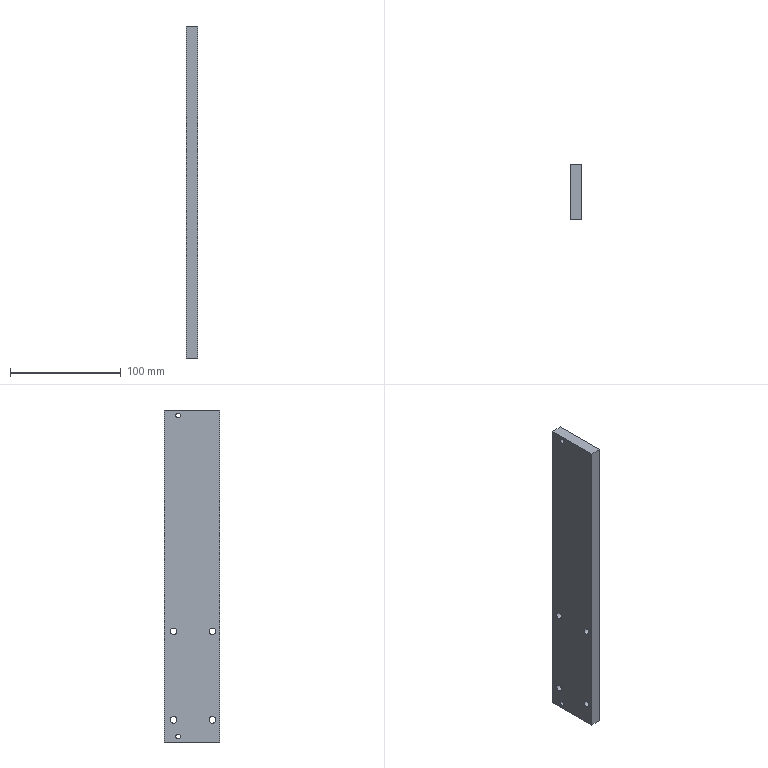Component | SolidWorks | ElectricalBoxAssembly2-1_GuidePlate-1 | 1 solid | 18 faces | box 10 x 50 x 300 mm | volume 148592 mm3 | cylinder 12 | plane 6 | commonest cylinder face diameters 6 x8 4.2 x4
build123d program:
from build123d import *

# Parameters (mm, degrees)
SKETCH1_W           = 300
SKETCH1_H           = 50
SKETCH1_R           = 3
BOSS_EXTRUDE1_DEPTH = 10
M5_TAPPED_HOLE1_D   = 4.2


with BuildPart() as part:
    # Sketch1 → Boss-Extrude1 (new body)
    with BuildSketch(Plane.XY):
        Rectangle(SKETCH1_W, SKETCH1_H)
        with Locations((130, 16.612)):
            Circle(SKETCH1_R, mode=Mode.SUBTRACT)
        with Locations((130, -18.388)):
            Circle(SKETCH1_R, mode=Mode.SUBTRACT)
        with Locations((50, 16.612)):
            Circle(SKETCH1_R, mode=Mode.SUBTRACT)
        with Locations((50, -18.388)):
            Circle(SKETCH1_R, mode=Mode.SUBTRACT)
    extrude(amount=BOSS_EXTRUDE1_DEPTH)

    # M5 Tapped Hole1 (through all)
    with Locations(Plane.XY.offset(10)):
        with Locations((-145, 12.5), (145, 12.5)):
            Hole(M5_TAPPED_HOLE1_D / 2)


solid = part.part

# Placed as in the assembly
solid = solid.moved(Location((745.468, 149.666, 1906.399), (0, 90, 0)))
STEP:
#1=COLOUR_RGB('',0.7922,0.8196,0.9333);
#2=FILL_AREA_STYLE_COLOUR('',#1);
#3=FILL_AREA_STYLE('',(#2));
#4=SURFACE_STYLE_FILL_AREA(#3);
#5=SURFACE_SIDE_STYLE('',(#4));
#6=SURFACE_STYLE_USAGE(.BOTH.,#5);
#7=PRESENTATION_STYLE_ASSIGNMENT((#6));
#8=CARTESIAN_POINT('',(29.349,6.384,80.846));
#9=VERTEX_POINT('',#8);
#10=CARTESIAN_POINT('',(29.349,6.384,80.681));
#11=VERTEX_POINT('',#10);
#12=CARTESIAN_POINT('',(29.349,6.384,80.764));
#13=DIRECTION('',(1.,-0.,0.));
#14=DIRECTION('',(0.,0.,-1.));
#15=AXIS2_PLACEMENT_3D('',#12,#13,#14);
#16=CIRCLE('',#15,0.08268);
#17=EDGE_CURVE('',#9,#11,#16,.T.);
#18=ORIENTED_EDGE('',*,*,#17,.F.);
#19=CARTESIAN_POINT('',(29.743,6.384,80.846));
#20=VERTEX_POINT('',#19);
#21=CARTESIAN_POINT('',(29.743,6.384,80.846));
#22=DIRECTION('',(1.,-0.,0.));
#23=VECTOR('',#22,39.37);
#24=LINE('',#21,#23);
#25=EDGE_CURVE('',#9,#20,#24,.T.);
#26=ORIENTED_EDGE('',*,*,#25,.T.);
#27=CARTESIAN_POINT('',(29.743,6.384,80.681));
#28=VERTEX_POINT('',#27);
#29=CARTESIAN_POINT('',(29.743,6.384,80.764));
#30=DIRECTION('',(1.,-0.,0.));
#31=DIRECTION('',(0.,0.,-1.));
#32=AXIS2_PLACEMENT_3D('',#29,#30,#31);
#33=CIRCLE('',#32,0.08268);
#34=EDGE_CURVE('',#20,#28,#33,.T.);
#35=ORIENTED_EDGE('',*,*,#34,.T.);
#36=CARTESIAN_POINT('',(29.743,6.384,80.681));
#37=DIRECTION('',(1.,-0.,0.));
#38=VECTOR('',#37,39.37);
#39=LINE('',#36,#38);
#40=EDGE_CURVE('',#11,#28,#39,.T.);
#41=ORIENTED_EDGE('',*,*,#40,.F.);
#42=EDGE_LOOP('',(#18,#26,#35,#41));
#43=FACE_OUTER_BOUND('',#42,.T.);
#44=CARTESIAN_POINT('',(29.743,6.384,80.764));
#45=DIRECTION('',(1.,-0.,0.));
#46=DIRECTION('',(0.,0.,-1.));
#47=AXIS2_PLACEMENT_3D('',#44,#45,#46);
#48=CYLINDRICAL_SURFACE('',#47,0.08268);
#49=ADVANCED_FACE('',(#43),#48,.F.);
#50=CARTESIAN_POINT('',(29.349,6.384,69.429));
#51=VERTEX_POINT('',#50);
#52=CARTESIAN_POINT('',(29.349,6.384,69.264));
#53=VERTEX_POINT('',#52);
#54=CARTESIAN_POINT('',(29.349,6.384,69.346));
#55=DIRECTION('',(1.,-0.,0.));
#56=DIRECTION('',(0.,0.,-1.));
#57=AXIS2_PLACEMENT_3D('',#54,#55,#56);
#58=CIRCLE('',#57,0.08268);
#59=EDGE_CURVE('',#51,#53,#58,.T.);
#60=ORIENTED_EDGE('',*,*,#59,.F.);
#61=CARTESIAN_POINT('',(29.743,6.384,69.429));
#62=VERTEX_POINT('',#61);
#63=CARTESIAN_POINT('',(29.743,6.384,69.429));
#64=DIRECTION('',(1.,-0.,0.));
#65=VECTOR('',#64,39.37);
#66=LINE('',#63,#65);
#67=EDGE_CURVE('',#51,#62,#66,.T.);
#68=ORIENTED_EDGE('',*,*,#67,.T.);
#69=CARTESIAN_POINT('',(29.743,6.384,69.264));
#70=VERTEX_POINT('',#69);
#71=CARTESIAN_POINT('',(29.743,6.384,69.346));
#72=DIRECTION('',(1.,-0.,0.));
#73=DIRECTION('',(0.,0.,-1.));
#74=AXIS2_PLACEMENT_3D('',#71,#72,#73);
#75=CIRCLE('',#74,0.08268);
#76=EDGE_CURVE('',#62,#70,#75,.T.);
#77=ORIENTED_EDGE('',*,*,#76,.T.);
#78=CARTESIAN_POINT('',(29.743,6.384,69.264));
#79=DIRECTION('',(1.,-0.,0.));
#80=VECTOR('',#79,39.37);
#81=LINE('',#78,#80);
#82=EDGE_CURVE('',#53,#70,#81,.T.);
#83=ORIENTED_EDGE('',*,*,#82,.F.);
#84=EDGE_LOOP('',(#60,#68,#77,#83));
#85=FACE_OUTER_BOUND('',#84,.T.);
#86=CARTESIAN_POINT('',(29.743,6.384,69.346));
#87=DIRECTION('',(1.,-0.,0.));
#88=DIRECTION('',(0.,0.,-1.));
#89=AXIS2_PLACEMENT_3D('',#86,#87,#88);
#90=CYLINDRICAL_SURFACE('',#89,0.08268);
#91=ADVANCED_FACE('',(#85),#90,.F.);
#92=CARTESIAN_POINT('',(29.743,5.168,73.205));
#93=VERTEX_POINT('',#92);
#94=CARTESIAN_POINT('',(29.743,5.168,72.968));
#95=VERTEX_POINT('',#94);
#96=CARTESIAN_POINT('',(29.743,5.168,73.087));
#97=DIRECTION('',(1.,-0.,0.));
#98=DIRECTION('',(0.,0.,-1.));
#99=AXIS2_PLACEMENT_3D('',#96,#97,#98);
#100=CIRCLE('',#99,0.1181);
#101=EDGE_CURVE('',#93,#95,#100,.T.);
#102=ORIENTED_EDGE('',*,*,#101,.T.);
#103=CARTESIAN_POINT('',(29.349,5.168,72.968));
#104=VERTEX_POINT('',#103);
#105=CARTESIAN_POINT('',(29.743,5.168,72.968));
#106=DIRECTION('',(-1.,0.,-0.));
#107=VECTOR('',#106,39.37);
#108=LINE('',#105,#107);
#109=EDGE_CURVE('',#95,#104,#108,.T.);
#110=ORIENTED_EDGE('',*,*,#109,.T.);
#111=CARTESIAN_POINT('',(29.349,5.168,73.205));
#112=VERTEX_POINT('',#111);
#113=CARTESIAN_POINT('',(29.349,5.168,73.087));
#114=DIRECTION('',(1.,-0.,0.));
#115=DIRECTION('',(0.,0.,-1.));
#116=AXIS2_PLACEMENT_3D('',#113,#114,#115);
#117=CIRCLE('',#116,0.1181);
#118=EDGE_CURVE('',#112,#104,#117,.T.);
#119=ORIENTED_EDGE('',*,*,#118,.F.);
#120=CARTESIAN_POINT('',(29.743,5.168,73.205));
#121=DIRECTION('',(-1.,0.,-0.));
#122=VECTOR('',#121,39.37);
#123=LINE('',#120,#122);
#124=EDGE_CURVE('',#93,#112,#123,.T.);
#125=ORIENTED_EDGE('',*,*,#124,.F.);
#126=EDGE_LOOP('',(#102,#110,#119,#125));
#127=FACE_OUTER_BOUND('',#126,.T.);
#128=CARTESIAN_POINT('',(29.743,5.168,73.087));
#129=DIRECTION('',(-1.,0.,-0.));
#130=DIRECTION('',(0.,0.,1.));
#131=AXIS2_PLACEMENT_3D('',#128,#129,#130);
#132=CYLINDRICAL_SURFACE('',#131,0.1181);
#133=ADVANCED_FACE('',(#127),#132,.F.);
#134=CARTESIAN_POINT('',(29.743,6.546,73.205));
#135=VERTEX_POINT('',#134);
#136=CARTESIAN_POINT('',(29.743,6.546,72.968));
#137=VERTEX_POINT('',#136);
#138=CARTESIAN_POINT('',(29.743,6.546,73.087));
#139=DIRECTION('',(1.,-0.,0.));
#140=DIRECTION('',(0.,0.,-1.));
#141=AXIS2_PLACEMENT_3D('',#138,#139,#140);
#142=CIRCLE('',#141,0.1181);
#143=EDGE_CURVE('',#135,#137,#142,.T.);
#144=ORIENTED_EDGE('',*,*,#143,.T.);
#145=CARTESIAN_POINT('',(29.349,6.546,72.968));
#146=VERTEX_POINT('',#145);
#147=CARTESIAN_POINT('',(29.743,6.546,72.968));
#148=DIRECTION('',(-1.,0.,-0.));
#149=VECTOR('',#148,39.37);
#150=LINE('',#147,#149);
#151=EDGE_CURVE('',#137,#146,#150,.T.);
#152=ORIENTED_EDGE('',*,*,#151,.T.);
#153=CARTESIAN_POINT('',(29.349,6.546,73.205));
#154=VERTEX_POINT('',#153);
#155=CARTESIAN_POINT('',(29.349,6.546,73.087));
#156=DIRECTION('',(1.,-0.,0.));
#157=DIRECTION('',(0.,0.,-1.));
#158=AXIS2_PLACEMENT_3D('',#155,#156,#157);
#159=CIRCLE('',#158,0.1181);
#160=EDGE_CURVE('',#154,#146,#159,.T.);
#161=ORIENTED_EDGE('',*,*,#160,.F.);
#162=CARTESIAN_POINT('',(29.743,6.546,73.205));
#163=DIRECTION('',(-1.,0.,-0.));
#164=VECTOR('',#163,39.37);
#165=LINE('',#162,#164);
#166=EDGE_CURVE('',#135,#154,#165,.T.);
#167=ORIENTED_EDGE('',*,*,#166,.F.);
#168=EDGE_LOOP('',(#144,#152,#161,#167));
#169=FACE_OUTER_BOUND('',#168,.T.);
#170=CARTESIAN_POINT('',(29.743,6.546,73.087));
#171=DIRECTION('',(-1.,0.,-0.));
#172=DIRECTION('',(0.,0.,1.));
#173=AXIS2_PLACEMENT_3D('',#170,#171,#172);
#174=CYLINDRICAL_SURFACE('',#173,0.1181);
#175=ADVANCED_FACE('',(#169),#174,.F.);
#176=CARTESIAN_POINT('',(29.743,5.168,70.055));
#177=VERTEX_POINT('',#176);
#178=CARTESIAN_POINT('',(29.743,5.168,69.819));
#179=VERTEX_POINT('',#178);
#180=CARTESIAN_POINT('',(29.743,5.168,69.937));
#181=DIRECTION('',(1.,-0.,0.));
#182=DIRECTION('',(0.,0.,-1.));
#183=AXIS2_PLACEMENT_3D('',#180,#181,#182);
#184=CIRCLE('',#183,0.1181);
#185=EDGE_CURVE('',#177,#179,#184,.T.);
#186=ORIENTED_EDGE('',*,*,#185,.T.);
#187=CARTESIAN_POINT('',(29.349,5.168,69.819));
#188=VERTEX_POINT('',#187);
#189=CARTESIAN_POINT('',(29.743,5.168,69.819));
#190=DIRECTION('',(-1.,0.,-0.));
#191=VECTOR('',#190,39.37);
#192=LINE('',#189,#191);
#193=EDGE_CURVE('',#179,#188,#192,.T.);
#194=ORIENTED_EDGE('',*,*,#193,.T.);
#195=CARTESIAN_POINT('',(29.349,5.168,70.055));
#196=VERTEX_POINT('',#195);
#197=CARTESIAN_POINT('',(29.349,5.168,69.937));
#198=DIRECTION('',(1.,-0.,0.));
#199=DIRECTION('',(0.,0.,-1.));
#200=AXIS2_PLACEMENT_3D('',#197,#198,#199);
#201=CIRCLE('',#200,0.1181);
#202=EDGE_CURVE('',#196,#188,#201,.T.);
#203=ORIENTED_EDGE('',*,*,#202,.F.);
#204=CARTESIAN_POINT('',(29.743,5.168,70.055));
#205=DIRECTION('',(-1.,0.,-0.));
#206=VECTOR('',#205,39.37);
#207=LINE('',#204,#206);
#208=EDGE_CURVE('',#177,#196,#207,.T.);
#209=ORIENTED_EDGE('',*,*,#208,.F.);
#210=EDGE_LOOP('',(#186,#194,#203,#209));
#211=FACE_OUTER_BOUND('',#210,.T.);
#212=CARTESIAN_POINT('',(29.743,5.168,69.937));
#213=DIRECTION('',(-1.,0.,-0.));
#214=DIRECTION('',(0.,0.,1.));
#215=AXIS2_PLACEMENT_3D('',#212,#213,#214);
#216=CYLINDRICAL_SURFACE('',#215,0.1181);
#217=ADVANCED_FACE('',(#211),#216,.F.);
#218=CARTESIAN_POINT('',(29.743,6.546,70.055));
#219=VERTEX_POINT('',#218);
#220=CARTESIAN_POINT('',(29.743,6.546,69.819));
#221=VERTEX_POINT('',#220);
#222=CARTESIAN_POINT('',(29.743,6.546,69.937));
#223=DIRECTION('',(1.,-0.,0.));
#224=DIRECTION('',(0.,0.,-1.));
#225=AXIS2_PLACEMENT_3D('',#222,#223,#224);
#226=CIRCLE('',#225,0.1181);
#227=EDGE_CURVE('',#219,#221,#226,.T.);
#228=ORIENTED_EDGE('',*,*,#227,.T.);
#229=CARTESIAN_POINT('',(29.349,6.546,69.819));
#230=VERTEX_POINT('',#229);
#231=CARTESIAN_POINT('',(29.743,6.546,69.819));
#232=DIRECTION('',(-1.,0.,-0.));
#233=VECTOR('',#232,39.37);
#234=LINE('',#231,#233);
#235=EDGE_CURVE('',#221,#230,#234,.T.);
#236=ORIENTED_EDGE('',*,*,#235,.T.);
#237=CARTESIAN_POINT('',(29.349,6.546,70.055));
#238=VERTEX_POINT('',#237);
#239=CARTESIAN_POINT('',(29.349,6.546,69.937));
#240=DIRECTION('',(1.,-0.,0.));
#241=DIRECTION('',(0.,0.,-1.));
#242=AXIS2_PLACEMENT_3D('',#239,#240,#241);
#243=CIRCLE('',#242,0.1181);
#244=EDGE_CURVE('',#238,#230,#243,.T.);
#245=ORIENTED_EDGE('',*,*,#244,.F.);
#246=CARTESIAN_POINT('',(29.743,6.546,70.055));
#247=DIRECTION('',(-1.,0.,-0.));
#248=VECTOR('',#247,39.37);
#249=LINE('',#246,#248);
#250=EDGE_CURVE('',#219,#238,#249,.T.);
#251=ORIENTED_EDGE('',*,*,#250,.F.);
#252=EDGE_LOOP('',(#228,#236,#245,#251));
#253=FACE_OUTER_BOUND('',#252,.T.);
#254=CARTESIAN_POINT('',(29.743,6.546,69.937));
#255=DIRECTION('',(-1.,0.,-0.));
#256=DIRECTION('',(0.,0.,1.));
#257=AXIS2_PLACEMENT_3D('',#254,#255,#256);
#258=CYLINDRICAL_SURFACE('',#257,0.1181);
#259=ADVANCED_FACE('',(#253),#258,.F.);
#260=CARTESIAN_POINT('',(29.743,6.384,80.764));
#261=DIRECTION('',(1.,-0.,0.));
#262=DIRECTION('',(0.,0.,-1.));
#263=AXIS2_PLACEMENT_3D('',#260,#261,#262);
#264=CIRCLE('',#263,0.08268);
#265=EDGE_CURVE('',#28,#20,#264,.T.);
#266=ORIENTED_EDGE('',*,*,#265,.F.);
#267=ORIENTED_EDGE('',*,*,#34,.F.);
#268=EDGE_LOOP('',(#266,#267));
#269=FACE_BOUND('',#268,.T.);
#270=CARTESIAN_POINT('',(29.743,6.384,69.346));
#271=DIRECTION('',(1.,-0.,0.));
#272=DIRECTION('',(0.,0.,-1.));
#273=AXIS2_PLACEMENT_3D('',#270,#271,#272);
#274=CIRCLE('',#273,0.08268);
#275=EDGE_CURVE('',#70,#62,#274,.T.);
#276=ORIENTED_EDGE('',*,*,#275,.F.);
#277=ORIENTED_EDGE('',*,*,#76,.F.);
#278=EDGE_LOOP('',(#276,#277));
#279=FACE_BOUND('',#278,.T.);
#280=ORIENTED_EDGE('',*,*,#143,.F.);
#281=CARTESIAN_POINT('',(29.743,6.546,73.087));
#282=DIRECTION('',(1.,-0.,0.));
#283=DIRECTION('',(0.,0.,-1.));
#284=AXIS2_PLACEMENT_3D('',#281,#282,#283);
#285=CIRCLE('',#284,0.1181);
#286=EDGE_CURVE('',#137,#135,#285,.T.);
#287=ORIENTED_EDGE('',*,*,#286,.F.);
#288=EDGE_LOOP('',(#280,#287));
#289=FACE_BOUND('',#288,.T.);
#290=ORIENTED_EDGE('',*,*,#227,.F.);
#291=CARTESIAN_POINT('',(29.743,6.546,69.937));
#292=DIRECTION('',(1.,-0.,0.));
#293=DIRECTION('',(0.,0.,-1.));
#294=AXIS2_PLACEMENT_3D('',#291,#292,#293);
#295=CIRCLE('',#294,0.1181);
#296=EDGE_CURVE('',#221,#219,#295,.T.);
#297=ORIENTED_EDGE('',*,*,#296,.F.);
#298=EDGE_LOOP('',(#290,#297));
#299=FACE_BOUND('',#298,.T.);
#300=CARTESIAN_POINT('',(29.743,4.908,69.15));
#301=VERTEX_POINT('',#300);
#302=CARTESIAN_POINT('',(29.743,6.877,69.15));
#303=VERTEX_POINT('',#302);
#304=CARTESIAN_POINT('',(29.743,6.877,69.15));
#305=DIRECTION('',(0.,1.,-0.));
#306=VECTOR('',#305,39.37);
#307=LINE('',#304,#306);
#308=EDGE_CURVE('',#301,#303,#307,.T.);
#309=ORIENTED_EDGE('',*,*,#308,.T.);
#310=CARTESIAN_POINT('',(29.743,6.877,80.961));
#311=VERTEX_POINT('',#310);
#312=CARTESIAN_POINT('',(29.743,6.877,80.961));
#313=DIRECTION('',(-0.,0.,1.));
#314=VECTOR('',#313,39.37);
#315=LINE('',#312,#314);
#316=EDGE_CURVE('',#303,#311,#315,.T.);
#317=ORIENTED_EDGE('',*,*,#316,.T.);
#318=CARTESIAN_POINT('',(29.743,4.908,80.961));
#319=VERTEX_POINT('',#318);
#320=CARTESIAN_POINT('',(29.743,6.877,80.961));
#321=DIRECTION('',(-0.,-1.,0.));
#322=VECTOR('',#321,39.37);
#323=LINE('',#320,#322);
#324=EDGE_CURVE('',#311,#319,#323,.T.);
#325=ORIENTED_EDGE('',*,*,#324,.T.);
#326=CARTESIAN_POINT('',(29.743,4.908,80.961));
#327=DIRECTION('',(0.,-0.,-1.));
#328=VECTOR('',#327,39.37);
#329=LINE('',#326,#328);
#330=EDGE_CURVE('',#319,#301,#329,.T.);
#331=ORIENTED_EDGE('',*,*,#330,.T.);
#332=EDGE_LOOP('',(#309,#317,#325,#331));
#333=FACE_OUTER_BOUND('',#332,.T.);
#334=ORIENTED_EDGE('',*,*,#185,.F.);
#335=CARTESIAN_POINT('',(29.743,5.168,69.937));
#336=DIRECTION('',(1.,-0.,0.));
#337=DIRECTION('',(0.,0.,-1.));
#338=AXIS2_PLACEMENT_3D('',#335,#336,#337);
#339=CIRCLE('',#338,0.1181);
#340=EDGE_CURVE('',#179,#177,#339,.T.);
#341=ORIENTED_EDGE('',*,*,#340,.F.);
#342=EDGE_LOOP('',(#334,#341));
#343=FACE_BOUND('',#342,.T.);
#344=ORIENTED_EDGE('',*,*,#101,.F.);
#345=CARTESIAN_POINT('',(29.743,5.168,73.087));
#346=DIRECTION('',(1.,-0.,0.));
#347=DIRECTION('',(0.,0.,-1.));
#348=AXIS2_PLACEMENT_3D('',#345,#346,#347);
#349=CIRCLE('',#348,0.1181);
#350=EDGE_CURVE('',#95,#93,#349,.T.);
#351=ORIENTED_EDGE('',*,*,#350,.F.);
#352=EDGE_LOOP('',(#344,#351));
#353=FACE_BOUND('',#352,.T.);
#354=CARTESIAN_POINT('',(29.743,5.892,75.055));
#355=DIRECTION('',(1.,-0.,0.));
#356=DIRECTION('',(0.,-0.,-1.));
#357=AXIS2_PLACEMENT_3D('',#354,#355,#356);
#358=PLANE('',#357);
#359=ADVANCED_FACE('',(#269,#279,#289,#299,#333,#343,#353),#358,.T.);
#360=CARTESIAN_POINT('',(29.349,6.384,80.764));
#361=DIRECTION('',(1.,-0.,0.));
#362=DIRECTION('',(0.,0.,-1.));
#363=AXIS2_PLACEMENT_3D('',#360,#361,#362);
#364=CIRCLE('',#363,0.08268);
#365=EDGE_CURVE('',#11,#9,#364,.T.);
#366=ORIENTED_EDGE('',*,*,#365,.T.);
#367=ORIENTED_EDGE('',*,*,#17,.T.);
#368=EDGE_LOOP('',(#366,#367));
#369=FACE_BOUND('',#368,.T.);
#370=CARTESIAN_POINT('',(29.349,6.384,69.346));
#371=DIRECTION('',(1.,-0.,0.));
#372=DIRECTION('',(0.,0.,-1.));
#373=AXIS2_PLACEMENT_3D('',#370,#371,#372);
#374=CIRCLE('',#373,0.08268);
#375=EDGE_CURVE('',#53,#51,#374,.T.);
#376=ORIENTED_EDGE('',*,*,#375,.T.);
#377=ORIENTED_EDGE('',*,*,#59,.T.);
#378=EDGE_LOOP('',(#376,#377));
#379=FACE_BOUND('',#378,.T.);
#380=CARTESIAN_POINT('',(29.349,4.908,69.15));
#381=VERTEX_POINT('',#380);
#382=CARTESIAN_POINT('',(29.349,6.877,69.15));
#383=VERTEX_POINT('',#382);
#384=CARTESIAN_POINT('',(29.349,6.877,69.15));
#385=DIRECTION('',(0.,1.,-0.));
#386=VECTOR('',#385,39.37);
#387=LINE('',#384,#386);
#388=EDGE_CURVE('',#381,#383,#387,.T.);
#389=ORIENTED_EDGE('',*,*,#388,.F.);
#390=CARTESIAN_POINT('',(29.349,4.908,80.961));
#391=VERTEX_POINT('',#390);
#392=CARTESIAN_POINT('',(29.349,4.908,80.961));
#393=DIRECTION('',(0.,-0.,-1.));
#394=VECTOR('',#393,39.37);
#395=LINE('',#392,#394);
#396=EDGE_CURVE('',#391,#381,#395,.T.);
#397=ORIENTED_EDGE('',*,*,#396,.F.);
#398=CARTESIAN_POINT('',(29.349,6.877,80.961));
#399=VERTEX_POINT('',#398);
#400=CARTESIAN_POINT('',(29.349,6.877,80.961));
#401=DIRECTION('',(-0.,-1.,0.));
#402=VECTOR('',#401,39.37);
#403=LINE('',#400,#402);
#404=EDGE_CURVE('',#399,#391,#403,.T.);
#405=ORIENTED_EDGE('',*,*,#404,.F.);
#406=CARTESIAN_POINT('',(29.349,6.877,80.961));
#407=DIRECTION('',(-0.,0.,1.));
#408=VECTOR('',#407,39.37);
#409=LINE('',#406,#408);
#410=EDGE_CURVE('',#383,#399,#409,.T.);
#411=ORIENTED_EDGE('',*,*,#410,.F.);
#412=EDGE_LOOP('',(#389,#397,#405,#411));
#413=FACE_OUTER_BOUND('',#412,.T.);
#414=ORIENTED_EDGE('',*,*,#244,.T.);
#415=CARTESIAN_POINT('',(29.349,6.546,69.937));
#416=DIRECTION('',(1.,-0.,0.));
#417=DIRECTION('',(0.,0.,-1.));
#418=AXIS2_PLACEMENT_3D('',#415,#416,#417);
#419=CIRCLE('',#418,0.1181);
#420=EDGE_CURVE('',#230,#238,#419,.T.);
#421=ORIENTED_EDGE('',*,*,#420,.T.);
#422=EDGE_LOOP('',(#414,#421));
#423=FACE_BOUND('',#422,.T.);
#424=ORIENTED_EDGE('',*,*,#202,.T.);
#425=CARTESIAN_POINT('',(29.349,5.168,69.937));
#426=DIRECTION('',(1.,-0.,0.));
#427=DIRECTION('',(0.,0.,-1.));
#428=AXIS2_PLACEMENT_3D('',#425,#426,#427);
#429=CIRCLE('',#428,0.1181);
#430=EDGE_CURVE('',#188,#196,#429,.T.);
#431=ORIENTED_EDGE('',*,*,#430,.T.);
#432=EDGE_LOOP('',(#424,#431));
#433=FACE_BOUND('',#432,.T.);
#434=ORIENTED_EDGE('',*,*,#160,.T.);
#435=CARTESIAN_POINT('',(29.349,6.546,73.087));
#436=DIRECTION('',(1.,-0.,0.));
#437=DIRECTION('',(0.,0.,-1.));
#438=AXIS2_PLACEMENT_3D('',#435,#436,#437);
#439=CIRCLE('',#438,0.1181);
#440=EDGE_CURVE('',#146,#154,#439,.T.);
#441=ORIENTED_EDGE('',*,*,#440,.T.);
#442=EDGE_LOOP('',(#434,#441));
#443=FACE_BOUND('',#442,.T.);
#444=ORIENTED_EDGE('',*,*,#118,.T.);
#445=CARTESIAN_POINT('',(29.349,5.168,73.087));
#446=DIRECTION('',(1.,-0.,0.));
#447=DIRECTION('',(0.,0.,-1.));
#448=AXIS2_PLACEMENT_3D('',#445,#446,#447);
#449=CIRCLE('',#448,0.1181);
#450=EDGE_CURVE('',#104,#112,#449,.T.);
#451=ORIENTED_EDGE('',*,*,#450,.T.);
#452=EDGE_LOOP('',(#444,#451));
#453=FACE_BOUND('',#452,.T.);
#454=CARTESIAN_POINT('',(29.349,5.892,75.055));
#455=DIRECTION('',(1.,-0.,0.));
#456=DIRECTION('',(0.,-0.,-1.));
#457=AXIS2_PLACEMENT_3D('',#454,#455,#456);
#458=PLANE('',#457);
#459=ADVANCED_FACE('',(#369,#379,#413,#423,#433,#443,#453),#458,.F.);
#460=ORIENTED_EDGE('',*,*,#388,.T.);
#461=CARTESIAN_POINT('',(29.743,6.877,69.15));
#462=DIRECTION('',(-1.,0.,-0.));
#463=VECTOR('',#462,39.37);
#464=LINE('',#461,#463);
#465=EDGE_CURVE('',#303,#383,#464,.T.);
#466=ORIENTED_EDGE('',*,*,#465,.F.);
#467=ORIENTED_EDGE('',*,*,#308,.F.);
#468=CARTESIAN_POINT('',(29.743,4.908,69.15));
#469=DIRECTION('',(-1.,0.,-0.));
#470=VECTOR('',#469,39.37);
#471=LINE('',#468,#470);
#472=EDGE_CURVE('',#301,#381,#471,.T.);
#473=ORIENTED_EDGE('',*,*,#472,.T.);
#474=EDGE_LOOP('',(#460,#466,#467,#473));
#475=FACE_OUTER_BOUND('',#474,.T.);
#476=CARTESIAN_POINT('',(29.743,6.877,69.15));
#477=DIRECTION('',(-0.,0.,1.));
#478=DIRECTION('',(1.,-0.,0.));
#479=AXIS2_PLACEMENT_3D('',#476,#477,#478);
#480=PLANE('',#479);
#481=ADVANCED_FACE('',(#475),#480,.F.);
#482=ORIENTED_EDGE('',*,*,#410,.T.);
#483=CARTESIAN_POINT('',(29.743,6.877,80.961));
#484=DIRECTION('',(-1.,0.,-0.));
#485=VECTOR('',#484,39.37);
#486=LINE('',#483,#485);
#487=EDGE_CURVE('',#311,#399,#486,.T.);
#488=ORIENTED_EDGE('',*,*,#487,.F.);
#489=ORIENTED_EDGE('',*,*,#316,.F.);
#490=ORIENTED_EDGE('',*,*,#465,.T.);
#491=EDGE_LOOP('',(#482,#488,#489,#490));
#492=FACE_OUTER_BOUND('',#491,.T.);
#493=CARTESIAN_POINT('',(29.743,6.877,80.961));
#494=DIRECTION('',(-0.,-1.,0.));
#495=DIRECTION('',(-1.,0.,-0.));
#496=AXIS2_PLACEMENT_3D('',#493,#494,#495);
#497=PLANE('',#496);
#498=ADVANCED_FACE('',(#492),#497,.F.);
#499=ORIENTED_EDGE('',*,*,#404,.T.);
#500=CARTESIAN_POINT('',(29.743,4.908,80.961));
#501=DIRECTION('',(-1.,0.,-0.));
#502=VECTOR('',#501,39.37);
#503=LINE('',#500,#502);
#504=EDGE_CURVE('',#319,#391,#503,.T.);
#505=ORIENTED_EDGE('',*,*,#504,.F.);
#506=ORIENTED_EDGE('',*,*,#324,.F.);
#507=ORIENTED_EDGE('',*,*,#487,.T.);
#508=EDGE_LOOP('',(#499,#505,#506,#507));
#509=FACE_OUTER_BOUND('',#508,.T.);
#510=CARTESIAN_POINT('',(29.743,6.877,80.961));
#511=DIRECTION('',(0.,-0.,-1.));
#512=DIRECTION('',(-1.,0.,-0.));
#513=AXIS2_PLACEMENT_3D('',#510,#511,#512);
#514=PLANE('',#513);
#515=ADVANCED_FACE('',(#509),#514,.F.);
#516=ORIENTED_EDGE('',*,*,#396,.T.);
#517=ORIENTED_EDGE('',*,*,#472,.F.);
#518=ORIENTED_EDGE('',*,*,#330,.F.);
#519=ORIENTED_EDGE('',*,*,#504,.T.);
#520=EDGE_LOOP('',(#516,#517,#518,#519));
#521=FACE_OUTER_BOUND('',#520,.T.);
#522=CARTESIAN_POINT('',(29.743,4.908,80.961));
#523=DIRECTION('',(0.,1.,-0.));
#524=DIRECTION('',(1.,-0.,0.));
#525=AXIS2_PLACEMENT_3D('',#522,#523,#524);
#526=PLANE('',#525);
#527=ADVANCED_FACE('',(#521),#526,.F.);
#528=ORIENTED_EDGE('',*,*,#235,.F.);
#529=ORIENTED_EDGE('',*,*,#296,.T.);
#530=ORIENTED_EDGE('',*,*,#250,.T.);
#531=ORIENTED_EDGE('',*,*,#420,.F.);
#532=EDGE_LOOP('',(#528,#529,#530,#531));
#533=FACE_OUTER_BOUND('',#532,.T.);
#534=CARTESIAN_POINT('',(29.743,6.546,69.937));
#535=DIRECTION('',(-1.,0.,-0.));
#536=DIRECTION('',(0.,0.,1.));
#537=AXIS2_PLACEMENT_3D('',#534,#535,#536);
#538=CYLINDRICAL_SURFACE('',#537,0.1181);
#539=ADVANCED_FACE('',(#533),#538,.F.);
#540=ORIENTED_EDGE('',*,*,#193,.F.);
#541=ORIENTED_EDGE('',*,*,#340,.T.);
#542=ORIENTED_EDGE('',*,*,#208,.T.);
#543=ORIENTED_EDGE('',*,*,#430,.F.);
#544=EDGE_LOOP('',(#540,#541,#542,#543));
#545=FACE_OUTER_BOUND('',#544,.T.);
#546=CARTESIAN_POINT('',(29.743,5.168,69.937));
#547=DIRECTION('',(-1.,0.,-0.));
#548=DIRECTION('',(0.,0.,1.));
#549=AXIS2_PLACEMENT_3D('',#546,#547,#548);
#550=CYLINDRICAL_SURFACE('',#549,0.1181);
#551=ADVANCED_FACE('',(#545),#550,.F.);
#552=ORIENTED_EDGE('',*,*,#151,.F.);
#553=ORIENTED_EDGE('',*,*,#286,.T.);
#554=ORIENTED_EDGE('',*,*,#166,.T.);
#555=ORIENTED_EDGE('',*,*,#440,.F.);
#556=EDGE_LOOP('',(#552,#553,#554,#555));
#557=FACE_OUTER_BOUND('',#556,.T.);
#558=CARTESIAN_POINT('',(29.743,6.546,73.087));
#559=DIRECTION('',(-1.,0.,-0.));
#560=DIRECTION('',(0.,0.,1.));
#561=AXIS2_PLACEMENT_3D('',#558,#559,#560);
#562=CYLINDRICAL_SURFACE('',#561,0.1181);
#563=ADVANCED_FACE('',(#557),#562,.F.);
#564=ORIENTED_EDGE('',*,*,#109,.F.);
#565=ORIENTED_EDGE('',*,*,#350,.T.);
#566=ORIENTED_EDGE('',*,*,#124,.T.);
#567=ORIENTED_EDGE('',*,*,#450,.F.);
#568=EDGE_LOOP('',(#564,#565,#566,#567));
#569=FACE_OUTER_BOUND('',#568,.T.);
#570=CARTESIAN_POINT('',(29.743,5.168,73.087));
#571=DIRECTION('',(-1.,0.,-0.));
#572=DIRECTION('',(0.,0.,1.));
#573=AXIS2_PLACEMENT_3D('',#570,#571,#572);
#574=CYLINDRICAL_SURFACE('',#573,0.1181);
#575=ADVANCED_FACE('',(#569),#574,.F.);
#576=ORIENTED_EDGE('',*,*,#67,.F.);
#577=ORIENTED_EDGE('',*,*,#375,.F.);
#578=ORIENTED_EDGE('',*,*,#82,.T.);
#579=ORIENTED_EDGE('',*,*,#275,.T.);
#580=EDGE_LOOP('',(#576,#577,#578,#579));
#581=FACE_OUTER_BOUND('',#580,.T.);
#582=CARTESIAN_POINT('',(29.743,6.384,69.346));
#583=DIRECTION('',(1.,-0.,0.));
#584=DIRECTION('',(0.,0.,-1.));
#585=AXIS2_PLACEMENT_3D('',#582,#583,#584);
#586=CYLINDRICAL_SURFACE('',#585,0.08268);
#587=ADVANCED_FACE('',(#581),#586,.F.);
#588=ORIENTED_EDGE('',*,*,#25,.F.);
#589=ORIENTED_EDGE('',*,*,#365,.F.);
#590=ORIENTED_EDGE('',*,*,#40,.T.);
#591=ORIENTED_EDGE('',*,*,#265,.T.);
#592=EDGE_LOOP('',(#588,#589,#590,#591));
#593=FACE_OUTER_BOUND('',#592,.T.);
#594=CARTESIAN_POINT('',(29.743,6.384,80.764));
#595=DIRECTION('',(1.,-0.,0.));
#596=DIRECTION('',(0.,0.,-1.));
#597=AXIS2_PLACEMENT_3D('',#594,#595,#596);
#598=CYLINDRICAL_SURFACE('',#597,0.08268);
#599=ADVANCED_FACE('',(#593),#598,.F.);
#600=CLOSED_SHELL('',(#49,#91,#133,#175,#217,#259,#359,#459,#481,#498,#515,#527,#539,#551,#563,#575,#587,#599));
#601=MANIFOLD_SOLID_BREP('',#600);
#602=STYLED_ITEM('',(#7),#601);
#603=PRESENTATION_LAYER_ASSIGNMENT('','',(#602));
#604=CARTESIAN_POINT('',(0.,0.,0.));
#605=DIRECTION('',(0.,0.,1.));
#606=DIRECTION('',(1.,0.,0.));
#607=AXIS2_PLACEMENT_3D('',#604,#605,#606);
#608=(LENGTH_UNIT()NAMED_UNIT(*)SI_UNIT($,.METRE.));
#609=LENGTH_MEASURE_WITH_UNIT(LENGTH_MEASURE(0.0254),#608);
#610=DIMENSIONAL_EXPONENTS(1.,0.,0.,0.,0.,0.,0.);
#611=(CONVERSION_BASED_UNIT('',#609)LENGTH_UNIT()NAMED_UNIT(#610));
#612=UNCERTAINTY_MEASURE_WITH_UNIT(LENGTH_MEASURE(0.00001),#611,'','');
#613=(NAMED_UNIT(*)PLANE_ANGLE_UNIT()SI_UNIT($,.RADIAN.));
#614=(NAMED_UNIT(*)SI_UNIT($,.STERADIAN.)SOLID_ANGLE_UNIT());
#615=(GEOMETRIC_REPRESENTATION_CONTEXT(3)GLOBAL_UNCERTAINTY_ASSIGNED_CONTEXT((#612))GLOBAL_UNIT_ASSIGNED_CONTEXT((#611,#613,#614))REPRESENTATION_CONTEXT('',''));
#616=ADVANCED_BREP_SHAPE_REPRESENTATION('',(#601,#607),#615);
#617=(LENGTH_UNIT()NAMED_UNIT(*)SI_UNIT($,.METRE.));
#618=LENGTH_MEASURE_WITH_UNIT(LENGTH_MEASURE(0.0254),#617);
#619=DIMENSIONAL_EXPONENTS(1.,0.,0.,0.,0.,0.,0.);
#620=(CONVERSION_BASED_UNIT('',#618)LENGTH_UNIT()NAMED_UNIT(#619));
#621=UNCERTAINTY_MEASURE_WITH_UNIT(LENGTH_MEASURE(0.00001),#620,'','');
#622=(NAMED_UNIT(*)PLANE_ANGLE_UNIT()SI_UNIT($,.RADIAN.));
#623=(NAMED_UNIT(*)SI_UNIT($,.STERADIAN.)SOLID_ANGLE_UNIT());
#624=(GEOMETRIC_REPRESENTATION_CONTEXT(3)GLOBAL_UNCERTAINTY_ASSIGNED_CONTEXT((#621))GLOBAL_UNIT_ASSIGNED_CONTEXT((#620,#622,#623))REPRESENTATION_CONTEXT('',''));
#625=MECHANICAL_DESIGN_GEOMETRIC_PRESENTATION_REPRESENTATION('',(#602),#624);